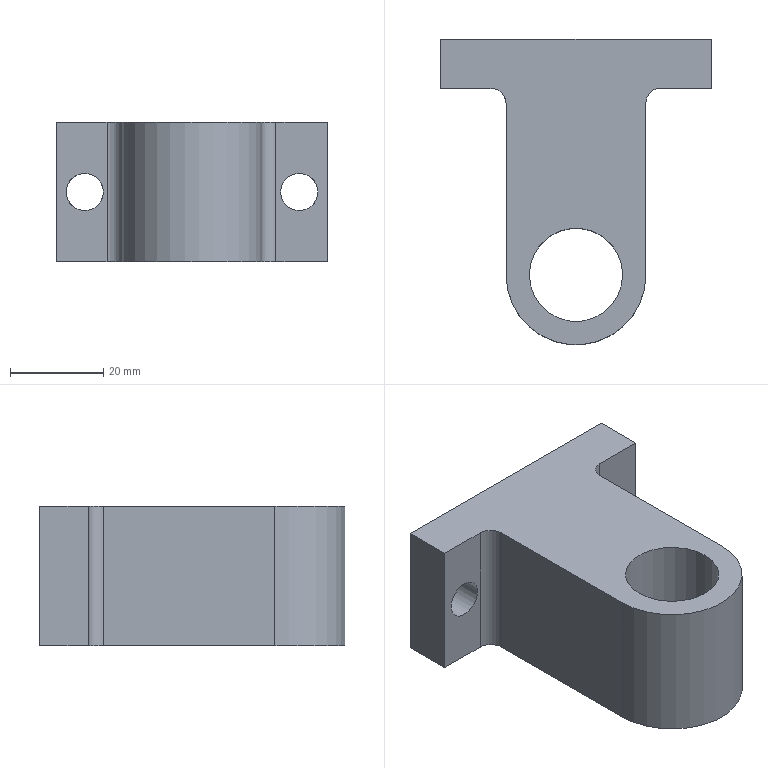Component | NX | YATAK | 1 solid | 15 faces | volume 54494 mm3 | plane 9 | cylinder 6 | commonest cylinder face diameters 8 x2 6.449 x1 6 x1 30 x1 20 x1